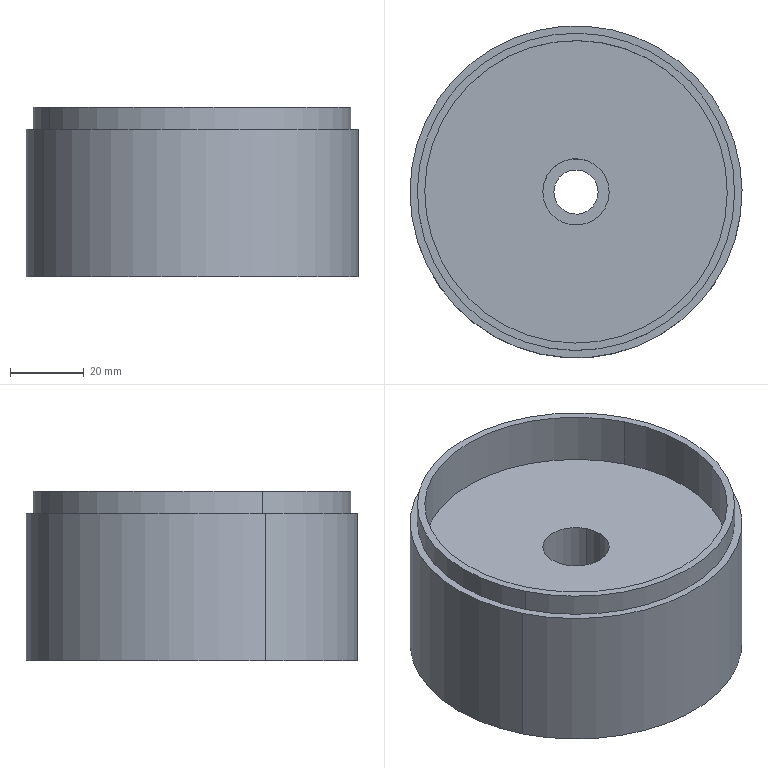Component | SolidWorks | g2-1 | 1 solid | 24 faces | box 90 x 90 x 46 mm | volume 54771 mm3 | cylinder 16 | plane 8 | commonest cylinder face diameters 86 x4 82 x4 12 x2 22 x2 18 x2 90 x2
build123d program:
from build123d import *
from build123d.topology import SkipClean

# Parameters (mm, degrees)
SKETCH1_R           = 45
SKETCH1_R_2         = 41
BOSS_EXTRUDE1_DEPTH = 20
BOSS_EXTRUDE2_START = 6
SKETCH2_R           = 43
SKETCH2_R_2         = 41
BOSS_EXTRUDE2_DEPTH = 6
SKETCH3_W           = 8
SKETCH3_H           = 4.784
SKETCH4_W           = 2
SKETCH4_H           = 36
BOSS_EXTRUDE3_START = 16
SKETCH5_R           = 11
SKETCH5_R_2         = 9
BOSS_EXTRUDE3_DEPTH = 16
BOSS_EXTRUDE4_START = 2
SKETCH6_R           = 11
SKETCH6_R_2         = 6
BOSS_EXTRUDE4_DEPTH = 2


with BuildPart() as part:
    # Sketch1 → Boss-Extrude1 (new, symmetric)
    with BuildSketch(Plane.XY):
        Circle(SKETCH1_R)
        Circle(SKETCH1_R_2, mode=Mode.SUBTRACT)
    extrude(amount=BOSS_EXTRUDE1_DEPTH, both=True)

    # Sketch2 → Boss-Extrude2 (add)
    with SkipClean():  # the faces are left unmerged after this step: merging them gives an invalid solid
        with BuildSketch(Plane(origin=(0, 0, -20), x_dir=(-1, 0, 0), z_dir=(0, 0, -1)).offset(BOSS_EXTRUDE2_START)):
            with Locations(Location((0, 0, 0), (0, 0, 180))):
                Circle(SKETCH2_R)
            Circle(SKETCH2_R_2, mode=Mode.SUBTRACT)
        extrude(amount=-BOSS_EXTRUDE2_DEPTH)

    # Sketch3 → Cut-Revolve2 (revolve, cut)
    with BuildSketch(Plane(origin=(0, 0, 0), x_dir=(0, 0, -1), z_dir=(1, 0, 0)), mode=Mode.PRIVATE) as cut_revolve2_sk:
        with Locations((-16, 40.608)):
            Rectangle(SKETCH3_W, SKETCH3_H)
    revolve(cut_revolve2_sk.sketch.rotate(Axis((0, 0, 50.051), (0, 0, -1)), 270), axis=Axis((0, 0, 50.051), (0, 0, -1)), mode=Mode.SUBTRACT)

    # Sketch4 → Revolve1 (revolve)
    with BuildSketch(Plane(origin=(0, 0, 0), x_dir=(0, 0, -1), z_dir=(1, 0, 0)), mode=Mode.PRIVATE) as revolve1_sk:
        with Locations((11, 27)):
            Rectangle(SKETCH4_W, SKETCH4_H)
    revolve(revolve1_sk.sketch.rotate(Axis((0, 0, 44.645), (0, 0, -1)), 270), axis=Axis((0, 0, 44.645), (0, 0, -1)))

    # Sketch5 → Boss-Extrude3 (add)
    with BuildSketch(Plane.XY.offset(-10).offset(BOSS_EXTRUDE3_START)):
        with Locations(Location((0, 0, 0), (0, 0, 180))):
            Circle(SKETCH5_R)
        Circle(SKETCH5_R_2, mode=Mode.SUBTRACT)
    extrude(amount=-BOSS_EXTRUDE3_DEPTH)

    # Sketch6 → Boss-Extrude4 (add)
    with BuildSketch(Plane.XY.offset(6).offset(BOSS_EXTRUDE4_START)):
        with Locations(Location((0, 0, 0), (0, 0, 180))):
            Circle(SKETCH6_R)
        Circle(SKETCH6_R_2, mode=Mode.SUBTRACT)
    extrude(amount=-BOSS_EXTRUDE4_DEPTH)


solid = part.part

# Placed as in the assembly
solid = solid.moved(Location((-15.928, -1.7, 148), (180, 0, 0)))
STEP:
#1=COLOUR_RGB('',0.7922,0.8196,0.9333);
#2=FILL_AREA_STYLE_COLOUR('',#1);
#3=FILL_AREA_STYLE('',(#2));
#4=SURFACE_STYLE_FILL_AREA(#3);
#5=SURFACE_SIDE_STYLE('',(#4));
#6=SURFACE_STYLE_USAGE(.BOTH.,#5);
#7=PRESENTATION_STYLE_ASSIGNMENT((#6));
#8=CARTESIAN_POINT('',(-0.4154,0.03795,5.512));
#9=VERTEX_POINT('',#8);
#10=CARTESIAN_POINT('',(-0.8387,-0.1718,5.512));
#11=VERTEX_POINT('',#10);
#12=CARTESIAN_POINT('',(-0.6271,-0.06694,5.512));
#13=DIRECTION('',(0.,0.,-1.));
#14=DIRECTION('',(-0.896,-0.444,0.));
#15=AXIS2_PLACEMENT_3D('',#12,#13,#14);
#16=CIRCLE('',#15,0.2362);
#17=EDGE_CURVE('',#9,#11,#16,.T.);
#18=ORIENTED_EDGE('',*,*,#17,.T.);
#19=CARTESIAN_POINT('',(-0.8387,-0.1718,5.591));
#20=VERTEX_POINT('',#19);
#21=CARTESIAN_POINT('',(-0.8387,-0.1718,5.512));
#22=DIRECTION('',(0.,0.,1.));
#23=VECTOR('',#22,39.37);
#24=LINE('',#21,#23);
#25=EDGE_CURVE('',#11,#20,#24,.T.);
#26=ORIENTED_EDGE('',*,*,#25,.T.);
#27=CARTESIAN_POINT('',(-0.4154,0.03795,5.591));
#28=VERTEX_POINT('',#27);
#29=CARTESIAN_POINT('',(-0.6271,-0.06694,5.591));
#30=DIRECTION('',(0.,0.,-1.));
#31=DIRECTION('',(-0.896,-0.444,0.));
#32=AXIS2_PLACEMENT_3D('',#29,#30,#31);
#33=CIRCLE('',#32,0.2362);
#34=EDGE_CURVE('',#28,#20,#33,.T.);
#35=ORIENTED_EDGE('',*,*,#34,.F.);
#36=CARTESIAN_POINT('',(-0.4154,0.03795,5.512));
#37=DIRECTION('',(0.,0.,1.));
#38=VECTOR('',#37,39.37);
#39=LINE('',#36,#38);
#40=EDGE_CURVE('',#9,#28,#39,.T.);
#41=ORIENTED_EDGE('',*,*,#40,.F.);
#42=EDGE_LOOP('',(#18,#26,#35,#41));
#43=FACE_OUTER_BOUND('',#42,.T.);
#44=CARTESIAN_POINT('',(-0.6271,-0.06694,5.512));
#45=DIRECTION('',(0.,0.,1.));
#46=DIRECTION('',(0.896,0.444,0.));
#47=AXIS2_PLACEMENT_3D('',#44,#45,#46);
#48=CYLINDRICAL_SURFACE('',#47,0.2362);
#49=ADVANCED_FACE('',(#43),#48,.F.);
#50=CARTESIAN_POINT('',(-1.015,-0.2592,5.512));
#51=VERTEX_POINT('',#50);
#52=CARTESIAN_POINT('',(-0.2391,0.1254,5.512));
#53=VERTEX_POINT('',#52);
#54=CARTESIAN_POINT('',(-0.6271,-0.06694,5.512));
#55=DIRECTION('',(0.,0.,-1.));
#56=DIRECTION('',(-0.896,-0.444,0.));
#57=AXIS2_PLACEMENT_3D('',#54,#55,#56);
#58=CIRCLE('',#57,0.4331);
#59=EDGE_CURVE('',#51,#53,#58,.T.);
#60=ORIENTED_EDGE('',*,*,#59,.F.);
#61=CARTESIAN_POINT('',(-1.015,-0.2592,6.22));
#62=VERTEX_POINT('',#61);
#63=CARTESIAN_POINT('',(-1.015,-0.2592,5.591));
#64=DIRECTION('',(0.,0.,1.));
#65=VECTOR('',#64,39.37);
#66=LINE('',#63,#65);
#67=EDGE_CURVE('',#51,#62,#66,.T.);
#68=ORIENTED_EDGE('',*,*,#67,.T.);
#69=CARTESIAN_POINT('',(-0.2391,0.1254,6.22));
#70=VERTEX_POINT('',#69);
#71=CARTESIAN_POINT('',(-0.6271,-0.06694,6.22));
#72=DIRECTION('',(0.,0.,-1.));
#73=DIRECTION('',(0.896,0.444,0.));
#74=AXIS2_PLACEMENT_3D('',#71,#72,#73);
#75=CIRCLE('',#74,0.4331);
#76=EDGE_CURVE('',#62,#70,#75,.T.);
#77=ORIENTED_EDGE('',*,*,#76,.T.);
#78=CARTESIAN_POINT('',(-0.2391,0.1254,5.591));
#79=DIRECTION('',(0.,0.,1.));
#80=VECTOR('',#79,39.37);
#81=LINE('',#78,#80);
#82=EDGE_CURVE('',#53,#70,#81,.T.);
#83=ORIENTED_EDGE('',*,*,#82,.F.);
#84=EDGE_LOOP('',(#60,#68,#77,#83));
#85=FACE_OUTER_BOUND('',#84,.T.);
#86=CARTESIAN_POINT('',(-0.6271,-0.06694,5.591));
#87=DIRECTION('',(0.,0.,1.));
#88=DIRECTION('',(0.896,0.444,0.));
#89=AXIS2_PLACEMENT_3D('',#86,#87,#88);
#90=CYLINDRICAL_SURFACE('',#89,0.4331);
#91=ADVANCED_FACE('',(#85),#90,.T.);
#92=CARTESIAN_POINT('',(-0.3096,0.0904,6.299));
#93=VERTEX_POINT('',#92);
#94=CARTESIAN_POINT('',(-0.9446,-0.2243,6.299));
#95=VERTEX_POINT('',#94);
#96=CARTESIAN_POINT('',(-0.6271,-0.06694,6.299));
#97=DIRECTION('',(0.,0.,-1.));
#98=DIRECTION('',(-0.896,-0.444,0.));
#99=AXIS2_PLACEMENT_3D('',#96,#97,#98);
#100=CIRCLE('',#99,0.3543);
#101=EDGE_CURVE('',#93,#95,#100,.T.);
#102=ORIENTED_EDGE('',*,*,#101,.F.);
#103=CARTESIAN_POINT('',(-0.3096,0.0904,5.591));
#104=VERTEX_POINT('',#103);
#105=CARTESIAN_POINT('',(-0.3096,0.0904,4.069));
#106=DIRECTION('',(0.,0.,-1.));
#107=VECTOR('',#106,39.37);
#108=LINE('',#105,#107);
#109=EDGE_CURVE('',#93,#104,#108,.T.);
#110=ORIENTED_EDGE('',*,*,#109,.T.);
#111=CARTESIAN_POINT('',(-0.9446,-0.2243,5.591));
#112=VERTEX_POINT('',#111);
#113=CARTESIAN_POINT('',(-0.6271,-0.06694,5.591));
#114=DIRECTION('',(0.,0.,1.));
#115=DIRECTION('',(-0.896,-0.444,0.));
#116=AXIS2_PLACEMENT_3D('',#113,#114,#115);
#117=CIRCLE('',#116,0.3543);
#118=EDGE_CURVE('',#112,#104,#117,.T.);
#119=ORIENTED_EDGE('',*,*,#118,.F.);
#120=CARTESIAN_POINT('',(-0.9446,-0.2243,4.069));
#121=DIRECTION('',(0.,0.,-1.));
#122=VECTOR('',#121,39.37);
#123=LINE('',#120,#122);
#124=EDGE_CURVE('',#95,#112,#123,.T.);
#125=ORIENTED_EDGE('',*,*,#124,.F.);
#126=EDGE_LOOP('',(#102,#110,#119,#125));
#127=FACE_OUTER_BOUND('',#126,.T.);
#128=CARTESIAN_POINT('',(-0.6271,-0.06694,4.069));
#129=DIRECTION('',(0.,0.,-1.));
#130=DIRECTION('',(-0.896,-0.444,0.));
#131=AXIS2_PLACEMENT_3D('',#128,#129,#130);
#132=CYLINDRICAL_SURFACE('',#131,0.3543);
#133=ADVANCED_FACE('',(#127),#132,.F.);
#134=CARTESIAN_POINT('',(0.8898,0.6848,5.354));
#135=VERTEX_POINT('',#134);
#136=CARTESIAN_POINT('',(-2.144,-0.8186,5.354));
#137=VERTEX_POINT('',#136);
#138=CARTESIAN_POINT('',(-0.6271,-0.06694,5.354));
#139=DIRECTION('',(0.,0.,-1.));
#140=DIRECTION('',(-0.896,-0.444,0.));
#141=AXIS2_PLACEMENT_3D('',#138,#139,#140);
#142=CIRCLE('',#141,1.693);
#143=EDGE_CURVE('',#135,#137,#142,.T.);
#144=ORIENTED_EDGE('',*,*,#143,.F.);
#145=CARTESIAN_POINT('',(0.8898,0.6848,5.039));
#146=VERTEX_POINT('',#145);
#147=CARTESIAN_POINT('',(0.8898,0.6848,3.856));
#148=DIRECTION('',(0.,0.,-1.));
#149=VECTOR('',#148,39.37);
#150=LINE('',#147,#149);
#151=EDGE_CURVE('',#135,#146,#150,.T.);
#152=ORIENTED_EDGE('',*,*,#151,.T.);
#153=CARTESIAN_POINT('',(-2.144,-0.8186,5.039));
#154=VERTEX_POINT('',#153);
#155=CARTESIAN_POINT('',(-0.6271,-0.06694,5.039));
#156=DIRECTION('',(0.,0.,-1.));
#157=DIRECTION('',(-0.896,-0.444,0.));
#158=AXIS2_PLACEMENT_3D('',#155,#156,#157);
#159=CIRCLE('',#158,1.693);
#160=EDGE_CURVE('',#146,#154,#159,.T.);
#161=ORIENTED_EDGE('',*,*,#160,.T.);
#162=CARTESIAN_POINT('',(-2.144,-0.8186,3.856));
#163=DIRECTION('',(0.,0.,-1.));
#164=VECTOR('',#163,39.37);
#165=LINE('',#162,#164);
#166=EDGE_CURVE('',#137,#154,#165,.T.);
#167=ORIENTED_EDGE('',*,*,#166,.F.);
#168=EDGE_LOOP('',(#144,#152,#161,#167));
#169=FACE_OUTER_BOUND('',#168,.T.);
#170=CARTESIAN_POINT('',(-0.6271,-0.06694,3.856));
#171=DIRECTION('',(0.,0.,-1.));
#172=DIRECTION('',(-0.896,-0.444,0.));
#173=AXIS2_PLACEMENT_3D('',#170,#171,#172);
#174=CYLINDRICAL_SURFACE('',#173,1.693);
#175=ADVANCED_FACE('',(#169),#174,.F.);
#176=CARTESIAN_POINT('',(0.8898,0.6848,6.85));
#177=VERTEX_POINT('',#176);
#178=CARTESIAN_POINT('',(-2.144,-0.8186,6.85));
#179=VERTEX_POINT('',#178);
#180=CARTESIAN_POINT('',(-0.6271,-0.06694,6.85));
#181=DIRECTION('',(0.,0.,1.));
#182=DIRECTION('',(0.896,0.444,0.));
#183=AXIS2_PLACEMENT_3D('',#180,#181,#182);
#184=CIRCLE('',#183,1.693);
#185=EDGE_CURVE('',#177,#179,#184,.T.);
#186=ORIENTED_EDGE('',*,*,#185,.F.);
#187=CARTESIAN_POINT('',(0.8898,0.6848,6.614));
#188=VERTEX_POINT('',#187);
#189=CARTESIAN_POINT('',(0.8898,0.6848,6.85));
#190=DIRECTION('',(0.,0.,-1.));
#191=VECTOR('',#190,39.37);
#192=LINE('',#189,#191);
#193=EDGE_CURVE('',#177,#188,#192,.T.);
#194=ORIENTED_EDGE('',*,*,#193,.T.);
#195=CARTESIAN_POINT('',(-2.144,-0.8186,6.614));
#196=VERTEX_POINT('',#195);
#197=CARTESIAN_POINT('',(-0.6271,-0.06694,6.614));
#198=DIRECTION('',(0.,0.,1.));
#199=DIRECTION('',(-0.896,-0.444,0.));
#200=AXIS2_PLACEMENT_3D('',#197,#198,#199);
#201=CIRCLE('',#200,1.693);
#202=EDGE_CURVE('',#188,#196,#201,.T.);
#203=ORIENTED_EDGE('',*,*,#202,.T.);
#204=CARTESIAN_POINT('',(-2.144,-0.8186,6.85));
#205=DIRECTION('',(0.,0.,-1.));
#206=VECTOR('',#205,39.37);
#207=LINE('',#204,#206);
#208=EDGE_CURVE('',#179,#196,#207,.T.);
#209=ORIENTED_EDGE('',*,*,#208,.F.);
#210=EDGE_LOOP('',(#186,#194,#203,#209));
#211=FACE_OUTER_BOUND('',#210,.T.);
#212=CARTESIAN_POINT('',(-0.6271,-0.06694,6.85));
#213=DIRECTION('',(0.,0.,-1.));
#214=DIRECTION('',(-0.896,-0.444,0.));
#215=AXIS2_PLACEMENT_3D('',#212,#213,#214);
#216=CYLINDRICAL_SURFACE('',#215,1.693);
#217=ADVANCED_FACE('',(#211),#216,.T.);
#218=CARTESIAN_POINT('',(-2.215,-0.8536,5.039));
#219=VERTEX_POINT('',#218);
#220=CARTESIAN_POINT('',(0.9603,0.7197,5.039));
#221=VERTEX_POINT('',#220);
#222=CARTESIAN_POINT('',(-0.6271,-0.06694,5.039));
#223=DIRECTION('',(0.,0.,-1.));
#224=DIRECTION('',(-0.896,-0.444,0.));
#225=AXIS2_PLACEMENT_3D('',#222,#223,#224);
#226=CIRCLE('',#225,1.772);
#227=EDGE_CURVE('',#219,#221,#226,.T.);
#228=ORIENTED_EDGE('',*,*,#227,.F.);
#229=CARTESIAN_POINT('',(-2.215,-0.8536,6.614));
#230=VERTEX_POINT('',#229);
#231=CARTESIAN_POINT('',(-2.215,-0.8536,5.039));
#232=DIRECTION('',(0.,0.,1.));
#233=VECTOR('',#232,39.37);
#234=LINE('',#231,#233);
#235=EDGE_CURVE('',#219,#230,#234,.T.);
#236=ORIENTED_EDGE('',*,*,#235,.T.);
#237=CARTESIAN_POINT('',(0.9603,0.7197,6.614));
#238=VERTEX_POINT('',#237);
#239=CARTESIAN_POINT('',(-0.6271,-0.06694,6.614));
#240=DIRECTION('',(0.,0.,-1.));
#241=DIRECTION('',(-0.896,-0.444,0.));
#242=AXIS2_PLACEMENT_3D('',#239,#240,#241);
#243=CIRCLE('',#242,1.772);
#244=EDGE_CURVE('',#230,#238,#243,.T.);
#245=ORIENTED_EDGE('',*,*,#244,.T.);
#246=CARTESIAN_POINT('',(0.9603,0.7197,5.039));
#247=DIRECTION('',(0.,0.,1.));
#248=VECTOR('',#247,39.37);
#249=LINE('',#246,#248);
#250=EDGE_CURVE('',#221,#238,#249,.T.);
#251=ORIENTED_EDGE('',*,*,#250,.F.);
#252=EDGE_LOOP('',(#228,#236,#245,#251));
#253=FACE_OUTER_BOUND('',#252,.T.);
#254=CARTESIAN_POINT('',(-0.6271,-0.06694,5.039));
#255=DIRECTION('',(0.,0.,1.));
#256=DIRECTION('',(0.896,0.444,0.));
#257=AXIS2_PLACEMENT_3D('',#254,#255,#256);
#258=CYLINDRICAL_SURFACE('',#257,1.772);
#259=ADVANCED_FACE('',(#253),#258,.T.);
#260=CARTESIAN_POINT('',(0.8192,0.6498,6.299));
#261=VERTEX_POINT('',#260);
#262=CARTESIAN_POINT('',(-2.073,-0.7837,6.299));
#263=VERTEX_POINT('',#262);
#264=CARTESIAN_POINT('',(-0.6271,-0.06694,6.299));
#265=DIRECTION('',(0.,0.,-1.));
#266=DIRECTION('',(-0.896,-0.444,0.));
#267=AXIS2_PLACEMENT_3D('',#264,#265,#266);
#268=CIRCLE('',#267,1.614);
#269=EDGE_CURVE('',#261,#263,#268,.T.);
#270=ORIENTED_EDGE('',*,*,#269,.T.);
#271=CARTESIAN_POINT('',(-2.073,-0.7837,6.85));
#272=VERTEX_POINT('',#271);
#273=CARTESIAN_POINT('',(-2.073,-0.7837,5.039));
#274=DIRECTION('',(0.,0.,1.));
#275=VECTOR('',#274,39.37);
#276=LINE('',#273,#275);
#277=EDGE_CURVE('',#263,#272,#276,.T.);
#278=ORIENTED_EDGE('',*,*,#277,.T.);
#279=CARTESIAN_POINT('',(0.8192,0.6498,6.85));
#280=VERTEX_POINT('',#279);
#281=CARTESIAN_POINT('',(-0.6271,-0.06694,6.85));
#282=DIRECTION('',(0.,0.,1.));
#283=DIRECTION('',(0.896,0.444,0.));
#284=AXIS2_PLACEMENT_3D('',#281,#282,#283);
#285=CIRCLE('',#284,1.614);
#286=EDGE_CURVE('',#272,#280,#285,.T.);
#287=ORIENTED_EDGE('',*,*,#286,.T.);
#288=CARTESIAN_POINT('',(0.8192,0.6498,5.039));
#289=DIRECTION('',(0.,0.,1.));
#290=VECTOR('',#289,39.37);
#291=LINE('',#288,#290);
#292=EDGE_CURVE('',#261,#280,#291,.T.);
#293=ORIENTED_EDGE('',*,*,#292,.F.);
#294=EDGE_LOOP('',(#270,#278,#287,#293));
#295=FACE_OUTER_BOUND('',#294,.T.);
#296=CARTESIAN_POINT('',(-0.6271,-0.06694,5.039));
#297=DIRECTION('',(0.,0.,1.));
#298=DIRECTION('',(0.896,0.444,0.));
#299=AXIS2_PLACEMENT_3D('',#296,#297,#298);
#300=CYLINDRICAL_SURFACE('',#299,1.614);
#301=ADVANCED_FACE('',(#295),#300,.F.);
#302=CARTESIAN_POINT('',(0.8192,0.6498,5.354));
#303=VERTEX_POINT('',#302);
#304=CARTESIAN_POINT('',(-2.073,-0.7837,5.354));
#305=VERTEX_POINT('',#304);
#306=CARTESIAN_POINT('',(-0.6271,-0.06694,5.354));
#307=DIRECTION('',(0.,0.,-1.));
#308=DIRECTION('',(-0.896,-0.444,0.));
#309=AXIS2_PLACEMENT_3D('',#306,#307,#308);
#310=CIRCLE('',#309,1.614);
#311=EDGE_CURVE('',#303,#305,#310,.T.);
#312=ORIENTED_EDGE('',*,*,#311,.T.);
#313=CARTESIAN_POINT('',(-2.073,-0.7837,6.22));
#314=VERTEX_POINT('',#313);
#315=CARTESIAN_POINT('',(-2.073,-0.7837,5.039));
#316=DIRECTION('',(0.,0.,1.));
#317=VECTOR('',#316,39.37);
#318=LINE('',#315,#317);
#319=EDGE_CURVE('',#305,#314,#318,.T.);
#320=ORIENTED_EDGE('',*,*,#319,.T.);
#321=CARTESIAN_POINT('',(0.8192,0.6498,6.22));
#322=VERTEX_POINT('',#321);
#323=CARTESIAN_POINT('',(-0.6271,-0.06694,6.22));
#324=DIRECTION('',(0.,0.,1.));
#325=DIRECTION('',(0.896,0.444,0.));
#326=AXIS2_PLACEMENT_3D('',#323,#324,#325);
#327=CIRCLE('',#326,1.614);
#328=EDGE_CURVE('',#314,#322,#327,.T.);
#329=ORIENTED_EDGE('',*,*,#328,.T.);
#330=CARTESIAN_POINT('',(0.8192,0.6498,5.039));
#331=DIRECTION('',(0.,0.,1.));
#332=VECTOR('',#331,39.37);
#333=LINE('',#330,#332);
#334=EDGE_CURVE('',#303,#322,#333,.T.);
#335=ORIENTED_EDGE('',*,*,#334,.F.);
#336=EDGE_LOOP('',(#312,#320,#329,#335));
#337=FACE_OUTER_BOUND('',#336,.T.);
#338=CARTESIAN_POINT('',(-0.6271,-0.06694,5.039));
#339=DIRECTION('',(0.,0.,1.));
#340=DIRECTION('',(0.896,0.444,0.));
#341=AXIS2_PLACEMENT_3D('',#338,#339,#340);
#342=CYLINDRICAL_SURFACE('',#341,1.614);
#343=ADVANCED_FACE('',(#337),#342,.F.);
#344=CARTESIAN_POINT('',(-0.6271,-0.06694,6.22));
#345=DIRECTION('',(0.,0.,1.));
#346=DIRECTION('',(0.896,0.444,0.));
#347=AXIS2_PLACEMENT_3D('',#344,#345,#346);
#348=CIRCLE('',#347,1.614);
#349=EDGE_CURVE('',#322,#314,#348,.T.);
#350=ORIENTED_EDGE('',*,*,#349,.F.);
#351=ORIENTED_EDGE('',*,*,#328,.F.);
#352=EDGE_LOOP('',(#350,#351));
#353=FACE_OUTER_BOUND('',#352,.T.);
#354=CARTESIAN_POINT('',(-0.6271,-0.06694,6.22));
#355=DIRECTION('',(0.,0.,-1.));
#356=DIRECTION('',(0.896,0.444,0.));
#357=AXIS2_PLACEMENT_3D('',#354,#355,#356);
#358=CIRCLE('',#357,0.4331);
#359=EDGE_CURVE('',#70,#62,#358,.T.);
#360=ORIENTED_EDGE('',*,*,#359,.F.);
#361=ORIENTED_EDGE('',*,*,#76,.F.);
#362=EDGE_LOOP('',(#360,#361));
#363=FACE_BOUND('',#362,.T.);
#364=CARTESIAN_POINT('',(-1.414,1.52,6.22));
#365=DIRECTION('',(0.,0.,1.));
#366=DIRECTION('',(0.896,0.444,0.));
#367=AXIS2_PLACEMENT_3D('',#364,#365,#366);
#368=PLANE('',#367);
#369=ADVANCED_FACE('',(#353,#363),#368,.F.);
#370=ORIENTED_EDGE('',*,*,#319,.F.);
#371=CARTESIAN_POINT('',(-0.6271,-0.06694,5.354));
#372=DIRECTION('',(0.,0.,-1.));
#373=DIRECTION('',(-0.896,-0.444,0.));
#374=AXIS2_PLACEMENT_3D('',#371,#372,#373);
#375=CIRCLE('',#374,1.614);
#376=EDGE_CURVE('',#305,#303,#375,.T.);
#377=ORIENTED_EDGE('',*,*,#376,.T.);
#378=ORIENTED_EDGE('',*,*,#334,.T.);
#379=ORIENTED_EDGE('',*,*,#349,.T.);
#380=EDGE_LOOP('',(#370,#377,#378,#379));
#381=FACE_OUTER_BOUND('',#380,.T.);
#382=CARTESIAN_POINT('',(-0.6271,-0.06694,5.039));
#383=DIRECTION('',(0.,0.,1.));
#384=DIRECTION('',(0.896,0.444,0.));
#385=AXIS2_PLACEMENT_3D('',#382,#383,#384);
#386=CYLINDRICAL_SURFACE('',#385,1.614);
#387=ADVANCED_FACE('',(#381),#386,.F.);
#388=ORIENTED_EDGE('',*,*,#277,.F.);
#389=CARTESIAN_POINT('',(-0.6271,-0.06694,6.299));
#390=DIRECTION('',(0.,0.,-1.));
#391=DIRECTION('',(-0.896,-0.444,0.));
#392=AXIS2_PLACEMENT_3D('',#389,#390,#391);
#393=CIRCLE('',#392,1.614);
#394=EDGE_CURVE('',#263,#261,#393,.T.);
#395=ORIENTED_EDGE('',*,*,#394,.T.);
#396=ORIENTED_EDGE('',*,*,#292,.T.);
#397=CARTESIAN_POINT('',(-0.6271,-0.06694,6.85));
#398=DIRECTION('',(0.,0.,1.));
#399=DIRECTION('',(0.896,0.444,0.));
#400=AXIS2_PLACEMENT_3D('',#397,#398,#399);
#401=CIRCLE('',#400,1.614);
#402=EDGE_CURVE('',#280,#272,#401,.T.);
#403=ORIENTED_EDGE('',*,*,#402,.T.);
#404=EDGE_LOOP('',(#388,#395,#396,#403));
#405=FACE_OUTER_BOUND('',#404,.T.);
#406=CARTESIAN_POINT('',(-0.6271,-0.06694,5.039));
#407=DIRECTION('',(0.,0.,1.));
#408=DIRECTION('',(0.896,0.444,0.));
#409=AXIS2_PLACEMENT_3D('',#406,#407,#408);
#410=CYLINDRICAL_SURFACE('',#409,1.614);
#411=ADVANCED_FACE('',(#405),#410,.F.);
#412=CARTESIAN_POINT('',(-0.6271,-0.06694,5.039));
#413=DIRECTION('',(0.,0.,-1.));
#414=DIRECTION('',(-0.896,-0.444,0.));
#415=AXIS2_PLACEMENT_3D('',#412,#413,#414);
#416=CIRCLE('',#415,1.772);
#417=EDGE_CURVE('',#221,#219,#416,.T.);
#418=ORIENTED_EDGE('',*,*,#417,.T.);
#419=ORIENTED_EDGE('',*,*,#227,.T.);
#420=EDGE_LOOP('',(#418,#419));
#421=FACE_OUTER_BOUND('',#420,.T.);
#422=CARTESIAN_POINT('',(-0.6271,-0.06694,5.039));
#423=DIRECTION('',(0.,0.,-1.));
#424=DIRECTION('',(-0.896,-0.444,0.));
#425=AXIS2_PLACEMENT_3D('',#422,#423,#424);
#426=CIRCLE('',#425,1.693);
#427=EDGE_CURVE('',#154,#146,#426,.T.);
#428=ORIENTED_EDGE('',*,*,#427,.F.);
#429=ORIENTED_EDGE('',*,*,#160,.F.);
#430=EDGE_LOOP('',(#428,#429));
#431=FACE_BOUND('',#430,.T.);
#432=CARTESIAN_POINT('',(-0.6271,-0.06694,5.039));
#433=DIRECTION('',(0.,0.,-1.));
#434=DIRECTION('',(-0.896,-0.444,0.));
#435=AXIS2_PLACEMENT_3D('',#432,#433,#434);
#436=PLANE('',#435);
#437=ADVANCED_FACE('',(#421,#431),#436,.T.);
#438=CARTESIAN_POINT('',(-0.6271,-0.06694,6.614));
#439=DIRECTION('',(0.,0.,-1.));
#440=DIRECTION('',(-0.896,-0.444,0.));
#441=AXIS2_PLACEMENT_3D('',#438,#439,#440);
#442=CIRCLE('',#441,1.772);
#443=EDGE_CURVE('',#238,#230,#442,.T.);
#444=ORIENTED_EDGE('',*,*,#443,.F.);
#445=ORIENTED_EDGE('',*,*,#244,.F.);
#446=EDGE_LOOP('',(#444,#445));
#447=FACE_OUTER_BOUND('',#446,.T.);
#448=CARTESIAN_POINT('',(-0.6271,-0.06694,6.614));
#449=DIRECTION('',(0.,0.,1.));
#450=DIRECTION('',(-0.896,-0.444,0.));
#451=AXIS2_PLACEMENT_3D('',#448,#449,#450);
#452=CIRCLE('',#451,1.693);
#453=EDGE_CURVE('',#196,#188,#452,.T.);
#454=ORIENTED_EDGE('',*,*,#453,.F.);
#455=ORIENTED_EDGE('',*,*,#202,.F.);
#456=EDGE_LOOP('',(#454,#455));
#457=FACE_BOUND('',#456,.T.);
#458=CARTESIAN_POINT('',(-0.6271,-0.06694,6.614));
#459=DIRECTION('',(0.,0.,-1.));
#460=DIRECTION('',(-0.896,-0.444,0.));
#461=AXIS2_PLACEMENT_3D('',#458,#459,#460);
#462=PLANE('',#461);
#463=ADVANCED_FACE('',(#447,#457),#462,.F.);
#464=ORIENTED_EDGE('',*,*,#235,.F.);
#465=ORIENTED_EDGE('',*,*,#417,.F.);
#466=ORIENTED_EDGE('',*,*,#250,.T.);
#467=ORIENTED_EDGE('',*,*,#443,.T.);
#468=EDGE_LOOP('',(#464,#465,#466,#467));
#469=FACE_OUTER_BOUND('',#468,.T.);
#470=CARTESIAN_POINT('',(-0.6271,-0.06694,5.039));
#471=DIRECTION('',(0.,0.,1.));
#472=DIRECTION('',(0.896,0.444,0.));
#473=AXIS2_PLACEMENT_3D('',#470,#471,#472);
#474=CYLINDRICAL_SURFACE('',#473,1.772);
#475=ADVANCED_FACE('',(#469),#474,.T.);
#476=CARTESIAN_POINT('',(-0.6271,-0.06694,6.85));
#477=DIRECTION('',(0.,0.,1.));
#478=DIRECTION('',(0.896,0.444,0.));
#479=AXIS2_PLACEMENT_3D('',#476,#477,#478);
#480=CIRCLE('',#479,1.693);
#481=EDGE_CURVE('',#179,#177,#480,.T.);
#482=ORIENTED_EDGE('',*,*,#481,.T.);
#483=ORIENTED_EDGE('',*,*,#185,.T.);
#484=EDGE_LOOP('',(#482,#483));
#485=FACE_OUTER_BOUND('',#484,.T.);
#486=ORIENTED_EDGE('',*,*,#402,.F.);
#487=ORIENTED_EDGE('',*,*,#286,.F.);
#488=EDGE_LOOP('',(#486,#487));
#489=FACE_BOUND('',#488,.T.);
#490=CARTESIAN_POINT('',(-0.6271,-0.06694,6.85));
#491=DIRECTION('',(0.,0.,1.));
#492=DIRECTION('',(0.896,0.444,0.));
#493=AXIS2_PLACEMENT_3D('',#490,#491,#492);
#494=PLANE('',#493);
#495=ADVANCED_FACE('',(#485,#489),#494,.T.);
#496=ORIENTED_EDGE('',*,*,#193,.F.);
#497=ORIENTED_EDGE('',*,*,#481,.F.);
#498=ORIENTED_EDGE('',*,*,#208,.T.);
#499=ORIENTED_EDGE('',*,*,#453,.T.);
#500=EDGE_LOOP('',(#496,#497,#498,#499));
#501=FACE_OUTER_BOUND('',#500,.T.);
#502=CARTESIAN_POINT('',(-0.6271,-0.06694,6.85));
#503=DIRECTION('',(0.,0.,-1.));
#504=DIRECTION('',(-0.896,-0.444,0.));
#505=AXIS2_PLACEMENT_3D('',#502,#503,#504);
#506=CYLINDRICAL_SURFACE('',#505,1.693);
#507=ADVANCED_FACE('',(#501),#506,.T.);
#508=ORIENTED_EDGE('',*,*,#311,.F.);
#509=ORIENTED_EDGE('',*,*,#376,.F.);
#510=EDGE_LOOP('',(#508,#509));
#511=FACE_BOUND('',#510,.T.);
#512=CARTESIAN_POINT('',(-0.6271,-0.06694,5.354));
#513=DIRECTION('',(0.,0.,-1.));
#514=DIRECTION('',(-0.896,-0.444,0.));
#515=AXIS2_PLACEMENT_3D('',#512,#513,#514);
#516=CIRCLE('',#515,1.693);
#517=EDGE_CURVE('',#137,#135,#516,.T.);
#518=ORIENTED_EDGE('',*,*,#517,.T.);
#519=ORIENTED_EDGE('',*,*,#143,.T.);
#520=EDGE_LOOP('',(#518,#519));
#521=FACE_OUTER_BOUND('',#520,.T.);
#522=CARTESIAN_POINT('',(-1.379,1.45,5.354));
#523=DIRECTION('',(0.,0.,-1.));
#524=DIRECTION('',(-0.896,-0.444,0.));
#525=AXIS2_PLACEMENT_3D('',#522,#523,#524);
#526=PLANE('',#525);
#527=ADVANCED_FACE('',(#511,#521),#526,.T.);
#528=ORIENTED_EDGE('',*,*,#151,.F.);
#529=ORIENTED_EDGE('',*,*,#517,.F.);
#530=ORIENTED_EDGE('',*,*,#166,.T.);
#531=ORIENTED_EDGE('',*,*,#427,.T.);
#532=EDGE_LOOP('',(#528,#529,#530,#531));
#533=FACE_OUTER_BOUND('',#532,.T.);
#534=CARTESIAN_POINT('',(-0.6271,-0.06694,3.856));
#535=DIRECTION('',(0.,0.,-1.));
#536=DIRECTION('',(-0.896,-0.444,0.));
#537=AXIS2_PLACEMENT_3D('',#534,#535,#536);
#538=CYLINDRICAL_SURFACE('',#537,1.693);
#539=ADVANCED_FACE('',(#533),#538,.F.);
#540=ORIENTED_EDGE('',*,*,#109,.F.);
#541=CARTESIAN_POINT('',(-0.6271,-0.06694,6.299));
#542=DIRECTION('',(0.,0.,-1.));
#543=DIRECTION('',(-0.896,-0.444,0.));
#544=AXIS2_PLACEMENT_3D('',#541,#542,#543);
#545=CIRCLE('',#544,0.3543);
#546=EDGE_CURVE('',#95,#93,#545,.T.);
#547=ORIENTED_EDGE('',*,*,#546,.F.);
#548=ORIENTED_EDGE('',*,*,#124,.T.);
#549=CARTESIAN_POINT('',(-0.6271,-0.06694,5.591));
#550=DIRECTION('',(0.,0.,1.));
#551=DIRECTION('',(-0.896,-0.444,0.));
#552=AXIS2_PLACEMENT_3D('',#549,#550,#551);
#553=CIRCLE('',#552,0.3543);
#554=EDGE_CURVE('',#104,#112,#553,.T.);
#555=ORIENTED_EDGE('',*,*,#554,.F.);
#556=EDGE_LOOP('',(#540,#547,#548,#555));
#557=FACE_OUTER_BOUND('',#556,.T.);
#558=CARTESIAN_POINT('',(-0.6271,-0.06694,4.069));
#559=DIRECTION('',(0.,0.,-1.));
#560=DIRECTION('',(-0.896,-0.444,0.));
#561=AXIS2_PLACEMENT_3D('',#558,#559,#560);
#562=CYLINDRICAL_SURFACE('',#561,0.3543);
#563=ADVANCED_FACE('',(#557),#562,.F.);
#564=ORIENTED_EDGE('',*,*,#269,.F.);
#565=ORIENTED_EDGE('',*,*,#394,.F.);
#566=EDGE_LOOP('',(#564,#565));
#567=FACE_OUTER_BOUND('',#566,.T.);
#568=ORIENTED_EDGE('',*,*,#546,.T.);
#569=ORIENTED_EDGE('',*,*,#101,.T.);
#570=EDGE_LOOP('',(#568,#569));
#571=FACE_BOUND('',#570,.T.);
#572=CARTESIAN_POINT('',(-1.414,1.52,6.299));
#573=DIRECTION('',(0.,0.,-1.));
#574=DIRECTION('',(-0.896,-0.444,0.));
#575=AXIS2_PLACEMENT_3D('',#572,#573,#574);
#576=PLANE('',#575);
#577=ADVANCED_FACE('',(#567,#571),#576,.F.);
#578=ORIENTED_EDGE('',*,*,#67,.F.);
#579=CARTESIAN_POINT('',(-0.6271,-0.06694,5.512));
#580=DIRECTION('',(0.,0.,-1.));
#581=DIRECTION('',(-0.896,-0.444,0.));
#582=AXIS2_PLACEMENT_3D('',#579,#580,#581);
#583=CIRCLE('',#582,0.4331);
#584=EDGE_CURVE('',#53,#51,#583,.T.);
#585=ORIENTED_EDGE('',*,*,#584,.F.);
#586=ORIENTED_EDGE('',*,*,#82,.T.);
#587=ORIENTED_EDGE('',*,*,#359,.T.);
#588=EDGE_LOOP('',(#578,#585,#586,#587));
#589=FACE_OUTER_BOUND('',#588,.T.);
#590=CARTESIAN_POINT('',(-0.6271,-0.06694,5.591));
#591=DIRECTION('',(0.,0.,1.));
#592=DIRECTION('',(0.896,0.444,0.));
#593=AXIS2_PLACEMENT_3D('',#590,#591,#592);
#594=CYLINDRICAL_SURFACE('',#593,0.4331);
#595=ADVANCED_FACE('',(#589),#594,.T.);
#596=ORIENTED_EDGE('',*,*,#34,.T.);
#597=CARTESIAN_POINT('',(-0.6271,-0.06694,5.591));
#598=DIRECTION('',(0.,0.,-1.));
#599=DIRECTION('',(-0.896,-0.444,0.));
#600=AXIS2_PLACEMENT_3D('',#597,#598,#599);
#601=CIRCLE('',#600,0.2362);
#602=EDGE_CURVE('',#20,#28,#601,.T.);
#603=ORIENTED_EDGE('',*,*,#602,.T.);
#604=EDGE_LOOP('',(#596,#603));
#605=FACE_BOUND('',#604,.T.);
#606=ORIENTED_EDGE('',*,*,#118,.T.);
#607=ORIENTED_EDGE('',*,*,#554,.T.);
#608=EDGE_LOOP('',(#606,#607));
#609=FACE_OUTER_BOUND('',#608,.T.);
#610=CARTESIAN_POINT('',(-0.6271,-0.06694,5.591));
#611=DIRECTION('',(0.,0.,-1.));
#612=DIRECTION('',(-0.896,-0.444,0.));
#613=AXIS2_PLACEMENT_3D('',#610,#611,#612);
#614=PLANE('',#613);
#615=ADVANCED_FACE('',(#605,#609),#614,.F.);
#616=ORIENTED_EDGE('',*,*,#584,.T.);
#617=ORIENTED_EDGE('',*,*,#59,.T.);
#618=EDGE_LOOP('',(#616,#617));
#619=FACE_OUTER_BOUND('',#618,.T.);
#620=ORIENTED_EDGE('',*,*,#17,.F.);
#621=CARTESIAN_POINT('',(-0.6271,-0.06694,5.512));
#622=DIRECTION('',(0.,0.,-1.));
#623=DIRECTION('',(-0.896,-0.444,0.));
#624=AXIS2_PLACEMENT_3D('',#621,#622,#623);
#625=CIRCLE('',#624,0.2362);
#626=EDGE_CURVE('',#11,#9,#625,.T.);
#627=ORIENTED_EDGE('',*,*,#626,.F.);
#628=EDGE_LOOP('',(#620,#627));
#629=FACE_BOUND('',#628,.T.);
#630=CARTESIAN_POINT('',(-0.6271,-0.06694,5.512));
#631=DIRECTION('',(0.,0.,-1.));
#632=DIRECTION('',(-0.896,-0.444,0.));
#633=AXIS2_PLACEMENT_3D('',#630,#631,#632);
#634=PLANE('',#633);
#635=ADVANCED_FACE('',(#619,#629),#634,.T.);
#636=ORIENTED_EDGE('',*,*,#25,.F.);
#637=ORIENTED_EDGE('',*,*,#626,.T.);
#638=ORIENTED_EDGE('',*,*,#40,.T.);
#639=ORIENTED_EDGE('',*,*,#602,.F.);
#640=EDGE_LOOP('',(#636,#637,#638,#639));
#641=FACE_OUTER_BOUND('',#640,.T.);
#642=CARTESIAN_POINT('',(-0.6271,-0.06694,5.512));
#643=DIRECTION('',(0.,0.,1.));
#644=DIRECTION('',(0.896,0.444,0.));
#645=AXIS2_PLACEMENT_3D('',#642,#643,#644);
#646=CYLINDRICAL_SURFACE('',#645,0.2362);
#647=ADVANCED_FACE('',(#641),#646,.F.);
#648=CLOSED_SHELL('',(#49,#91,#133,#175,#217,#259,#301,#343,#369,#387,#411,#437,#463,#475,#495,#507,#527,#539,#563,#577,#595,#615,#635,#647));
#649=MANIFOLD_SOLID_BREP('',#648);
#650=STYLED_ITEM('',(#7),#649);
#651=(LENGTH_UNIT()NAMED_UNIT(*)SI_UNIT($,.METRE.));
#652=LENGTH_MEASURE_WITH_UNIT(LENGTH_MEASURE(0.0254),#651);
#653=DIMENSIONAL_EXPONENTS(1.,0.,0.,0.,0.,0.,0.);
#654=(CONVERSION_BASED_UNIT('',#652)LENGTH_UNIT()NAMED_UNIT(#653));
#655=UNCERTAINTY_MEASURE_WITH_UNIT(LENGTH_MEASURE(0.00001),#654,'','');
#656=(NAMED_UNIT(*)PLANE_ANGLE_UNIT()SI_UNIT($,.RADIAN.));
#657=(NAMED_UNIT(*)SI_UNIT($,.STERADIAN.)SOLID_ANGLE_UNIT());
#658=(GEOMETRIC_REPRESENTATION_CONTEXT(3)GLOBAL_UNCERTAINTY_ASSIGNED_CONTEXT((#655))GLOBAL_UNIT_ASSIGNED_CONTEXT((#654,#656,#657))REPRESENTATION_CONTEXT('',''));
#659=MECHANICAL_DESIGN_GEOMETRIC_PRESENTATION_REPRESENTATION('',(#650),#658);
#660=CARTESIAN_POINT('',(0.,0.,0.));
#661=DIRECTION('',(0.,0.,1.));
#662=DIRECTION('',(1.,0.,0.));
#663=AXIS2_PLACEMENT_3D('',#660,#661,#662);
#664=(LENGTH_UNIT()NAMED_UNIT(*)SI_UNIT($,.METRE.));
#665=LENGTH_MEASURE_WITH_UNIT(LENGTH_MEASURE(0.0254),#664);
#666=DIMENSIONAL_EXPONENTS(1.,0.,0.,0.,0.,0.,0.);
#667=(CONVERSION_BASED_UNIT('',#665)LENGTH_UNIT()NAMED_UNIT(#666));
#668=UNCERTAINTY_MEASURE_WITH_UNIT(LENGTH_MEASURE(0.00001),#667,'','');
#669=(NAMED_UNIT(*)PLANE_ANGLE_UNIT()SI_UNIT($,.RADIAN.));
#670=(NAMED_UNIT(*)SI_UNIT($,.STERADIAN.)SOLID_ANGLE_UNIT());
#671=(GEOMETRIC_REPRESENTATION_CONTEXT(3)GLOBAL_UNCERTAINTY_ASSIGNED_CONTEXT((#668))GLOBAL_UNIT_ASSIGNED_CONTEXT((#667,#669,#670))REPRESENTATION_CONTEXT('',''));
#672=ADVANCED_BREP_SHAPE_REPRESENTATION('',(#649,#663),#671);
#673=PRESENTATION_LAYER_ASSIGNMENT('','',(#650));